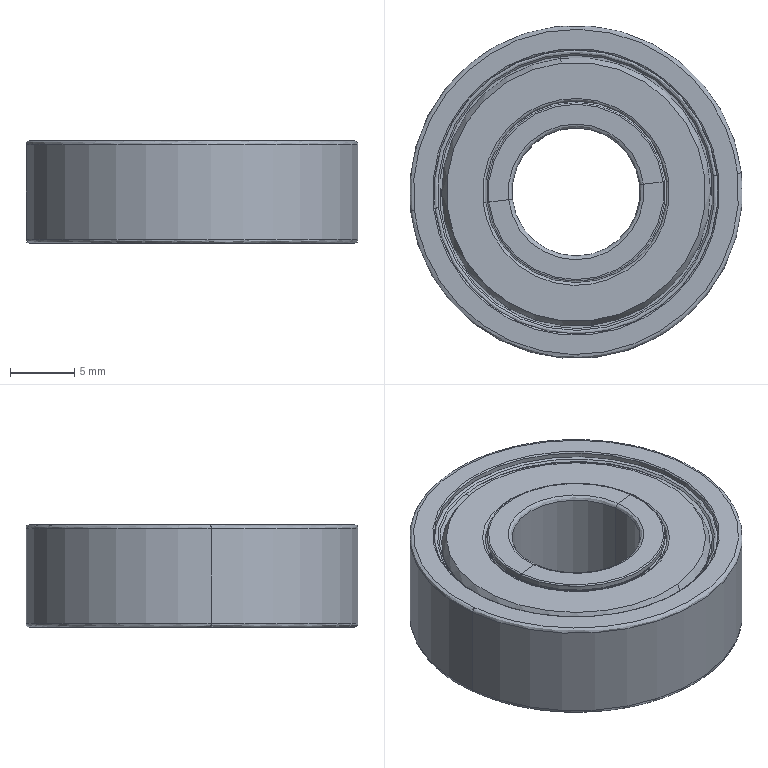Component | SolidWorks | 170423A4-IdlerAssembly5-10_170423A4-BAY6000ZZ-2 | 1 solid | 142 faces | volume 2960 mm3 | spline 52 | cone 48 | cylinder 32 | plane 10 | commonest cylinder face diameters 22.2 x4 14.2 x4 14.6 x4 20.8 x4 14.8 x4 13.3 x4 13.9 x4 26 x2